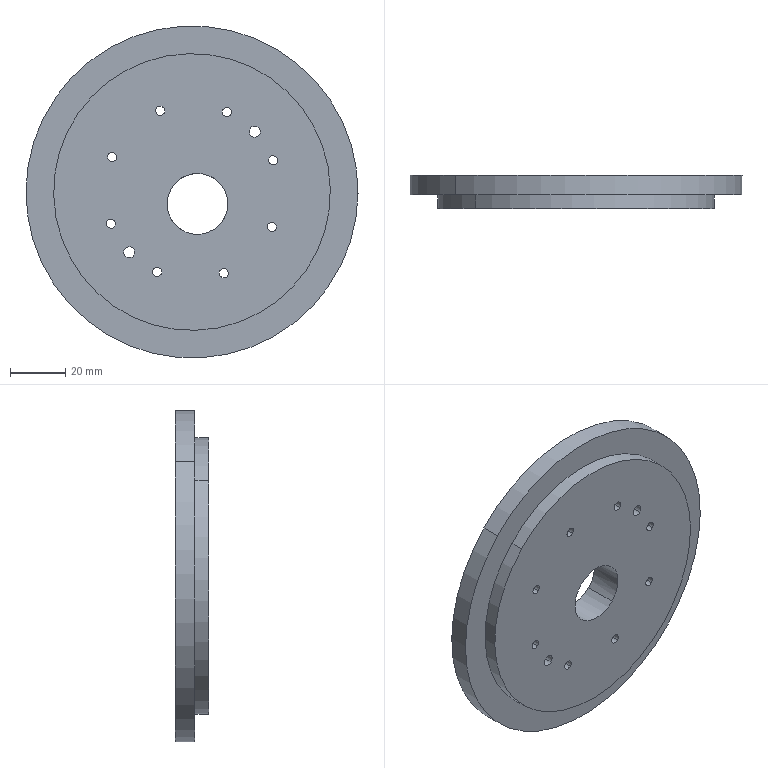Component | SolidWorks | PushRodMotorPlatform-1 | 1 solid | 29 faces | box 120 x 12 x 120 mm | volume 112754 mm3 | cylinder 26 | plane 3 | commonest cylinder face diameters 3.3 x16 4 x4 22 x2 100 x2 120 x2
build123d program:
from build123d import *

# Parameters (mm, degrees)
SKETCH1_2_R             = 60
SKETCH1_2_R_2           = 1.65
SKETCH1_2_R_3           = 2
BOSS_EXTRUDE1_DEPTH     = 12
SKETCH2_R               = 60
SKETCH2_R_2             = 50
CUT_EXTRUDE1_2_DEPTH    = 5
CUT_EXTRUDE1_DEPTH      = 320.099
CUT_EXTRUDE1_DEPTH_BACK = 320.099
SKETCH1_R               = 11


with BuildPart() as part:
    # Sketch1_2 → Boss-Extrude1 (new body)
    with BuildSketch(Plane.XY):
        with Locations((90, 221.39)):
            Circle(SKETCH1_2_R)
        with Locations((118.509, 234.787)):
            Circle(SKETCH1_2_R_2, mode=Mode.SUBTRACT)
        with Locations((119.632, 210.705)):
            Circle(SKETCH1_2_R_2, mode=Mode.SUBTRACT)
        with Locations((103.398, 192.881)):
            Circle(SKETCH1_2_R_2, mode=Mode.SUBTRACT)
        with Locations((91.468, 189.924)):
            Circle(SKETCH1_2_R_3, mode=Mode.SUBTRACT)
        with Locations((79.315, 191.757)):
            Circle(SKETCH1_2_R_2, mode=Mode.SUBTRACT)
        with Locations((61.491, 207.992)):
            Circle(SKETCH1_2_R_2, mode=Mode.SUBTRACT)
        with Locations((60.368, 232.075)):
            Circle(SKETCH1_2_R_2, mode=Mode.SUBTRACT)
        with Locations((76.602, 249.899)):
            Circle(SKETCH1_2_R_2, mode=Mode.SUBTRACT)
        with Locations((88.532, 252.856)):
            Circle(SKETCH1_2_R_3, mode=Mode.SUBTRACT)
        with Locations((100.685, 251.022)):
            Circle(SKETCH1_2_R_2, mode=Mode.SUBTRACT)
    extrude(amount=BOSS_EXTRUDE1_DEPTH)

    # Sketch2 → Cut-Extrude1_2 (cut)
    with BuildSketch(Plane(origin=(0, 0, 0), x_dir=(-1, 0, 0), z_dir=(0, 0, -1))):
        with Locations((-90, 221.39)):
            Circle(SKETCH2_R)
        with Locations((-90, 221.39)):
            Circle(SKETCH2_R_2, mode=Mode.SUBTRACT)
    extrude(amount=-CUT_EXTRUDE1_2_DEPTH, mode=Mode.SUBTRACT)

    # Sketch1 → Cut-Extrude1 (cut, two sides: drawn at the far end of the back side and taken through both)
    with BuildSketch(Plane.XY.offset(-CUT_EXTRUDE1_DEPTH_BACK)):
        with Locations((85.6, 219.613)):
            Circle(SKETCH1_R)
    extrude(amount=CUT_EXTRUDE1_DEPTH + CUT_EXTRUDE1_DEPTH_BACK, mode=Mode.SUBTRACT)


solid = part.part

# Placed as in the assembly
solid = solid.moved(Location((499.474, 964, -2315.533), (-90, 0, -136.538)))
STEP:
#1=COLOUR_RGB('',0.7922,0.8196,0.9333);
#2=FILL_AREA_STYLE_COLOUR('',#1);
#3=FILL_AREA_STYLE('',(#2));
#4=SURFACE_STYLE_FILL_AREA(#3);
#5=SURFACE_SIDE_STYLE('',(#4));
#6=SURFACE_STYLE_USAGE(.BOTH.,#5);
#7=PRESENTATION_STYLE_ASSIGNMENT((#6));
#8=CARTESIAN_POINT('',(23.48,37.953,-82.867));
#9=VERTEX_POINT('',#8);
#10=CARTESIAN_POINT('',(22.851,37.953,-82.271));
#11=VERTEX_POINT('',#10);
#12=CARTESIAN_POINT('',(23.48,37.953,-82.867));
#13=CARTESIAN_POINT('',(23.441,37.953,-82.908));
#14=CARTESIAN_POINT('',(23.395,37.953,-82.941));
#15=CARTESIAN_POINT('',(23.29,37.953,-82.988));
#16=CARTESIAN_POINT('',(23.235,37.953,-83.));
#17=CARTESIAN_POINT('',(23.12,37.953,-83.003));
#18=CARTESIAN_POINT('',(23.064,37.953,-82.994));
#19=CARTESIAN_POINT('',(22.957,37.953,-82.953));
#20=CARTESIAN_POINT('',(22.91,37.953,-82.923));
#21=CARTESIAN_POINT('',(22.826,37.953,-82.844));
#22=CARTESIAN_POINT('',(22.794,37.953,-82.798));
#23=CARTESIAN_POINT('',(22.747,37.953,-82.693));
#24=CARTESIAN_POINT('',(22.734,37.953,-82.638));
#25=CARTESIAN_POINT('',(22.731,37.953,-82.523));
#26=CARTESIAN_POINT('',(22.741,37.953,-82.468));
#27=CARTESIAN_POINT('',(22.782,37.953,-82.36));
#28=CARTESIAN_POINT('',(22.812,37.953,-82.313));
#29=CARTESIAN_POINT('',(22.851,37.953,-82.271));
#30=B_SPLINE_CURVE_WITH_KNOTS('',3,(#12,#13,#14,#15,#16,#17,#18,#19,#20,#21,#22,#23,#24,#25,#26,#27,#28,#29),.UNSPECIFIED.,.F.,.F.,(4,2,2,2,2,2,2,2,4),(0.5,0.5625,0.625,0.6875,0.75,0.8125,0.875,0.9375,1.),.UNSPECIFIED.);
#31=EDGE_CURVE('',#9,#11,#30,.T.);
#32=ORIENTED_EDGE('',*,*,#31,.F.);
#33=CARTESIAN_POINT('',(23.48,38.425,-82.867));
#34=VERTEX_POINT('',#33);
#35=CARTESIAN_POINT('',(23.48,37.953,-82.867));
#36=DIRECTION('',(-0.,1.,0.));
#37=VECTOR('',#36,39.37);
#38=LINE('',#35,#37);
#39=EDGE_CURVE('',#9,#34,#38,.T.);
#40=ORIENTED_EDGE('',*,*,#39,.T.);
#41=CARTESIAN_POINT('',(22.851,38.425,-82.271));
#42=VERTEX_POINT('',#41);
#43=CARTESIAN_POINT('',(23.166,38.425,-82.569));
#44=DIRECTION('',(-0.,1.,0.));
#45=DIRECTION('',(-0.7258,0.,0.6879));
#46=AXIS2_PLACEMENT_3D('',#43,#44,#45);
#47=CIRCLE('',#46,0.4331);
#48=EDGE_CURVE('',#34,#42,#47,.T.);
#49=ORIENTED_EDGE('',*,*,#48,.T.);
#50=CARTESIAN_POINT('',(22.851,37.953,-82.271));
#51=DIRECTION('',(-0.,1.,0.));
#52=VECTOR('',#51,39.37);
#53=LINE('',#50,#52);
#54=EDGE_CURVE('',#11,#42,#53,.T.);
#55=ORIENTED_EDGE('',*,*,#54,.F.);
#56=EDGE_LOOP('',(#32,#40,#49,#55));
#57=FACE_OUTER_BOUND('',#56,.T.);
#58=CARTESIAN_POINT('',(23.166,37.953,-82.569));
#59=DIRECTION('',(-0.,1.,0.));
#60=DIRECTION('',(-0.7258,0.,0.6879));
#61=AXIS2_PLACEMENT_3D('',#58,#59,#60);
#62=CYLINDRICAL_SURFACE('',#61,0.4331);
#63=ADVANCED_FACE('',(#57),#62,.F.);
#64=CARTESIAN_POINT('',(24.517,38.15,-83.753));
#65=VERTEX_POINT('',#64);
#66=CARTESIAN_POINT('',(21.659,38.15,-81.045));
#67=VERTEX_POINT('',#66);
#68=CARTESIAN_POINT('',(23.088,38.15,-82.399));
#69=DIRECTION('',(0.,-1.,-0.));
#70=DIRECTION('',(0.7258,0.,-0.6879));
#71=AXIS2_PLACEMENT_3D('',#68,#69,#70);
#72=CIRCLE('',#71,1.969);
#73=EDGE_CURVE('',#65,#67,#72,.T.);
#74=ORIENTED_EDGE('',*,*,#73,.T.);
#75=CARTESIAN_POINT('',(21.659,37.953,-81.045));
#76=VERTEX_POINT('',#75);
#77=CARTESIAN_POINT('',(21.659,38.15,-81.045));
#78=DIRECTION('',(0.,-1.,-0.));
#79=VECTOR('',#78,39.37);
#80=LINE('',#77,#79);
#81=EDGE_CURVE('',#67,#76,#80,.T.);
#82=ORIENTED_EDGE('',*,*,#81,.T.);
#83=CARTESIAN_POINT('',(24.517,37.953,-83.753));
#84=VERTEX_POINT('',#83);
#85=CARTESIAN_POINT('',(23.088,37.953,-82.399));
#86=DIRECTION('',(0.,-1.,-0.));
#87=DIRECTION('',(0.7258,0.,-0.6879));
#88=AXIS2_PLACEMENT_3D('',#85,#86,#87);
#89=CIRCLE('',#88,1.969);
#90=EDGE_CURVE('',#84,#76,#89,.T.);
#91=ORIENTED_EDGE('',*,*,#90,.F.);
#92=CARTESIAN_POINT('',(24.517,38.15,-83.753));
#93=DIRECTION('',(0.,-1.,-0.));
#94=VECTOR('',#93,39.37);
#95=LINE('',#92,#94);
#96=EDGE_CURVE('',#65,#84,#95,.T.);
#97=ORIENTED_EDGE('',*,*,#96,.F.);
#98=EDGE_LOOP('',(#74,#82,#91,#97));
#99=FACE_OUTER_BOUND('',#98,.T.);
#100=CARTESIAN_POINT('',(23.088,38.15,-82.399));
#101=DIRECTION('',(0.,-1.,-0.));
#102=DIRECTION('',(0.7258,0.,-0.6879));
#103=AXIS2_PLACEMENT_3D('',#100,#101,#102);
#104=CYLINDRICAL_SURFACE('',#103,1.969);
#105=ADVANCED_FACE('',(#99),#104,.T.);
#106=CARTESIAN_POINT('',(23.632,38.425,-81.308));
#107=VERTEX_POINT('',#106);
#108=CARTESIAN_POINT('',(23.538,38.425,-81.218));
#109=VERTEX_POINT('',#108);
#110=CARTESIAN_POINT('',(23.585,38.425,-81.263));
#111=DIRECTION('',(-0.,1.,0.));
#112=DIRECTION('',(-0.7258,0.,0.6879));
#113=AXIS2_PLACEMENT_3D('',#110,#111,#112);
#114=CIRCLE('',#113,0.06496);
#115=EDGE_CURVE('',#107,#109,#114,.T.);
#116=ORIENTED_EDGE('',*,*,#115,.T.);
#117=CARTESIAN_POINT('',(23.538,37.953,-81.218));
#118=VERTEX_POINT('',#117);
#119=CARTESIAN_POINT('',(23.538,38.425,-81.218));
#120=DIRECTION('',(0.,-1.,-0.));
#121=VECTOR('',#120,39.37);
#122=LINE('',#119,#121);
#123=EDGE_CURVE('',#109,#118,#122,.T.);
#124=ORIENTED_EDGE('',*,*,#123,.T.);
#125=CARTESIAN_POINT('',(23.632,37.953,-81.308));
#126=VERTEX_POINT('',#125);
#127=CARTESIAN_POINT('',(23.585,37.953,-81.263));
#128=DIRECTION('',(-0.,1.,0.));
#129=DIRECTION('',(-0.7258,0.,0.6879));
#130=AXIS2_PLACEMENT_3D('',#127,#128,#129);
#131=CIRCLE('',#130,0.06496);
#132=EDGE_CURVE('',#126,#118,#131,.T.);
#133=ORIENTED_EDGE('',*,*,#132,.F.);
#134=CARTESIAN_POINT('',(23.632,38.425,-81.308));
#135=DIRECTION('',(0.,-1.,-0.));
#136=VECTOR('',#135,39.37);
#137=LINE('',#134,#136);
#138=EDGE_CURVE('',#107,#126,#137,.T.);
#139=ORIENTED_EDGE('',*,*,#138,.F.);
#140=EDGE_LOOP('',(#116,#124,#133,#139));
#141=FACE_OUTER_BOUND('',#140,.T.);
#142=CARTESIAN_POINT('',(23.585,38.425,-81.263));
#143=DIRECTION('',(0.,-1.,-0.));
#144=DIRECTION('',(0.7258,0.,-0.6879));
#145=AXIS2_PLACEMENT_3D('',#142,#143,#144);
#146=CYLINDRICAL_SURFACE('',#145,0.06496);
#147=ADVANCED_FACE('',(#141),#146,.F.);
#148=CARTESIAN_POINT('',(24.039,38.425,-81.594));
#149=VERTEX_POINT('',#148);
#150=CARTESIAN_POINT('',(23.925,38.425,-81.485));
#151=VERTEX_POINT('',#150);
#152=CARTESIAN_POINT('',(23.982,38.425,-81.54));
#153=DIRECTION('',(-0.,1.,0.));
#154=DIRECTION('',(-0.7258,0.,0.6879));
#155=AXIS2_PLACEMENT_3D('',#152,#153,#154);
#156=CIRCLE('',#155,0.07874);
#157=EDGE_CURVE('',#149,#151,#156,.T.);
#158=ORIENTED_EDGE('',*,*,#157,.T.);
#159=CARTESIAN_POINT('',(23.925,37.953,-81.485));
#160=VERTEX_POINT('',#159);
#161=CARTESIAN_POINT('',(23.925,38.425,-81.485));
#162=DIRECTION('',(0.,-1.,-0.));
#163=VECTOR('',#162,39.37);
#164=LINE('',#161,#163);
#165=EDGE_CURVE('',#151,#160,#164,.T.);
#166=ORIENTED_EDGE('',*,*,#165,.T.);
#167=CARTESIAN_POINT('',(24.039,37.953,-81.594));
#168=VERTEX_POINT('',#167);
#169=CARTESIAN_POINT('',(23.982,37.953,-81.54));
#170=DIRECTION('',(-0.,1.,0.));
#171=DIRECTION('',(-0.7258,0.,0.6879));
#172=AXIS2_PLACEMENT_3D('',#169,#170,#171);
#173=CIRCLE('',#172,0.07874);
#174=EDGE_CURVE('',#168,#160,#173,.T.);
#175=ORIENTED_EDGE('',*,*,#174,.F.);
#176=CARTESIAN_POINT('',(24.039,38.425,-81.594));
#177=DIRECTION('',(0.,-1.,-0.));
#178=VECTOR('',#177,39.37);
#179=LINE('',#176,#178);
#180=EDGE_CURVE('',#149,#168,#179,.T.);
#181=ORIENTED_EDGE('',*,*,#180,.F.);
#182=EDGE_LOOP('',(#158,#166,#175,#181));
#183=FACE_OUTER_BOUND('',#182,.T.);
#184=CARTESIAN_POINT('',(23.982,38.425,-81.54));
#185=DIRECTION('',(0.,-1.,-0.));
#186=DIRECTION('',(0.7258,0.,-0.6879));
#187=AXIS2_PLACEMENT_3D('',#184,#185,#186);
#188=CYLINDRICAL_SURFACE('',#187,0.07874);
#189=ADVANCED_FACE('',(#183),#188,.F.);
#190=CARTESIAN_POINT('',(24.29,38.425,-81.992));
#191=VERTEX_POINT('',#190);
#192=CARTESIAN_POINT('',(24.196,38.425,-81.902));
#193=VERTEX_POINT('',#192);
#194=CARTESIAN_POINT('',(24.243,38.425,-81.947));
#195=DIRECTION('',(-0.,1.,0.));
#196=DIRECTION('',(-0.7258,0.,0.6879));
#197=AXIS2_PLACEMENT_3D('',#194,#195,#196);
#198=CIRCLE('',#197,0.06496);
#199=EDGE_CURVE('',#191,#193,#198,.T.);
#200=ORIENTED_EDGE('',*,*,#199,.T.);
#201=CARTESIAN_POINT('',(24.196,37.953,-81.902));
#202=VERTEX_POINT('',#201);
#203=CARTESIAN_POINT('',(24.196,38.425,-81.902));
#204=DIRECTION('',(0.,-1.,-0.));
#205=VECTOR('',#204,39.37);
#206=LINE('',#203,#205);
#207=EDGE_CURVE('',#193,#202,#206,.T.);
#208=ORIENTED_EDGE('',*,*,#207,.T.);
#209=CARTESIAN_POINT('',(24.29,37.953,-81.992));
#210=VERTEX_POINT('',#209);
#211=CARTESIAN_POINT('',(24.243,37.953,-81.947));
#212=DIRECTION('',(-0.,1.,0.));
#213=DIRECTION('',(-0.7258,0.,0.6879));
#214=AXIS2_PLACEMENT_3D('',#211,#212,#213);
#215=CIRCLE('',#214,0.06496);
#216=EDGE_CURVE('',#210,#202,#215,.T.);
#217=ORIENTED_EDGE('',*,*,#216,.F.);
#218=CARTESIAN_POINT('',(24.29,38.425,-81.992));
#219=DIRECTION('',(0.,-1.,-0.));
#220=VECTOR('',#219,39.37);
#221=LINE('',#218,#220);
#222=EDGE_CURVE('',#191,#210,#221,.T.);
#223=ORIENTED_EDGE('',*,*,#222,.F.);
#224=EDGE_LOOP('',(#200,#208,#217,#223));
#225=FACE_OUTER_BOUND('',#224,.T.);
#226=CARTESIAN_POINT('',(24.243,38.425,-81.947));
#227=DIRECTION('',(0.,-1.,-0.));
#228=DIRECTION('',(0.7258,0.,-0.6879));
#229=AXIS2_PLACEMENT_3D('',#226,#227,#228);
#230=CYLINDRICAL_SURFACE('',#229,0.06496);
#231=ADVANCED_FACE('',(#225),#230,.F.);
#232=CARTESIAN_POINT('',(24.271,38.425,-82.941));
#233=VERTEX_POINT('',#232);
#234=CARTESIAN_POINT('',(24.177,38.425,-82.851));
#235=VERTEX_POINT('',#234);
#236=CARTESIAN_POINT('',(24.224,38.425,-82.896));
#237=DIRECTION('',(-0.,1.,0.));
#238=DIRECTION('',(-0.7258,0.,0.6879));
#239=AXIS2_PLACEMENT_3D('',#236,#237,#238);
#240=CIRCLE('',#239,0.06496);
#241=EDGE_CURVE('',#233,#235,#240,.T.);
#242=ORIENTED_EDGE('',*,*,#241,.T.);
#243=CARTESIAN_POINT('',(24.177,37.953,-82.851));
#244=VERTEX_POINT('',#243);
#245=CARTESIAN_POINT('',(24.177,38.425,-82.851));
#246=DIRECTION('',(0.,-1.,-0.));
#247=VECTOR('',#246,39.37);
#248=LINE('',#245,#247);
#249=EDGE_CURVE('',#235,#244,#248,.T.);
#250=ORIENTED_EDGE('',*,*,#249,.T.);
#251=CARTESIAN_POINT('',(24.271,37.953,-82.941));
#252=VERTEX_POINT('',#251);
#253=CARTESIAN_POINT('',(24.224,37.953,-82.896));
#254=DIRECTION('',(-0.,1.,0.));
#255=DIRECTION('',(-0.7258,0.,0.6879));
#256=AXIS2_PLACEMENT_3D('',#253,#254,#255);
#257=CIRCLE('',#256,0.06496);
#258=EDGE_CURVE('',#252,#244,#257,.T.);
#259=ORIENTED_EDGE('',*,*,#258,.F.);
#260=CARTESIAN_POINT('',(24.271,38.425,-82.941));
#261=DIRECTION('',(0.,-1.,-0.));
#262=VECTOR('',#261,39.37);
#263=LINE('',#260,#262);
#264=EDGE_CURVE('',#233,#252,#263,.T.);
#265=ORIENTED_EDGE('',*,*,#264,.F.);
#266=EDGE_LOOP('',(#242,#250,#259,#265));
#267=FACE_OUTER_BOUND('',#266,.T.);
#268=CARTESIAN_POINT('',(24.224,38.425,-82.896));
#269=DIRECTION('',(0.,-1.,-0.));
#270=DIRECTION('',(0.7258,0.,-0.6879));
#271=AXIS2_PLACEMENT_3D('',#268,#269,#270);
#272=CYLINDRICAL_SURFACE('',#271,0.06496);
#273=ADVANCED_FACE('',(#267),#272,.F.);
#274=CARTESIAN_POINT('',(23.587,38.425,-83.599));
#275=VERTEX_POINT('',#274);
#276=CARTESIAN_POINT('',(23.493,38.425,-83.509));
#277=VERTEX_POINT('',#276);
#278=CARTESIAN_POINT('',(23.54,38.425,-83.554));
#279=DIRECTION('',(-0.,1.,0.));
#280=DIRECTION('',(-0.7258,0.,0.6879));
#281=AXIS2_PLACEMENT_3D('',#278,#279,#280);
#282=CIRCLE('',#281,0.06496);
#283=EDGE_CURVE('',#275,#277,#282,.T.);
#284=ORIENTED_EDGE('',*,*,#283,.T.);
#285=CARTESIAN_POINT('',(23.493,37.953,-83.509));
#286=VERTEX_POINT('',#285);
#287=CARTESIAN_POINT('',(23.493,38.425,-83.509));
#288=DIRECTION('',(0.,-1.,-0.));
#289=VECTOR('',#288,39.37);
#290=LINE('',#287,#289);
#291=EDGE_CURVE('',#277,#286,#290,.T.);
#292=ORIENTED_EDGE('',*,*,#291,.T.);
#293=CARTESIAN_POINT('',(23.587,37.953,-83.599));
#294=VERTEX_POINT('',#293);
#295=CARTESIAN_POINT('',(23.54,37.953,-83.554));
#296=DIRECTION('',(-0.,1.,0.));
#297=DIRECTION('',(-0.7258,0.,0.6879));
#298=AXIS2_PLACEMENT_3D('',#295,#296,#297);
#299=CIRCLE('',#298,0.06496);
#300=EDGE_CURVE('',#294,#286,#299,.T.);
#301=ORIENTED_EDGE('',*,*,#300,.F.);
#302=CARTESIAN_POINT('',(23.587,38.425,-83.599));
#303=DIRECTION('',(0.,-1.,-0.));
#304=VECTOR('',#303,39.37);
#305=LINE('',#302,#304);
#306=EDGE_CURVE('',#275,#294,#305,.T.);
#307=ORIENTED_EDGE('',*,*,#306,.F.);
#308=EDGE_LOOP('',(#284,#292,#301,#307));
#309=FACE_OUTER_BOUND('',#308,.T.);
#310=CARTESIAN_POINT('',(23.54,38.425,-83.554));
#311=DIRECTION('',(0.,-1.,-0.));
#312=DIRECTION('',(0.7258,0.,-0.6879));
#313=AXIS2_PLACEMENT_3D('',#310,#311,#312);
#314=CYLINDRICAL_SURFACE('',#313,0.06496);
#315=ADVANCED_FACE('',(#309),#314,.F.);
#316=CARTESIAN_POINT('',(22.638,38.425,-83.58));
#317=VERTEX_POINT('',#316);
#318=CARTESIAN_POINT('',(22.544,38.425,-83.49));
#319=VERTEX_POINT('',#318);
#320=CARTESIAN_POINT('',(22.591,38.425,-83.535));
#321=DIRECTION('',(-0.,1.,0.));
#322=DIRECTION('',(-0.7258,0.,0.6879));
#323=AXIS2_PLACEMENT_3D('',#320,#321,#322);
#324=CIRCLE('',#323,0.06496);
#325=EDGE_CURVE('',#317,#319,#324,.T.);
#326=ORIENTED_EDGE('',*,*,#325,.T.);
#327=CARTESIAN_POINT('',(22.544,37.953,-83.49));
#328=VERTEX_POINT('',#327);
#329=CARTESIAN_POINT('',(22.544,38.425,-83.49));
#330=DIRECTION('',(0.,-1.,-0.));
#331=VECTOR('',#330,39.37);
#332=LINE('',#329,#331);
#333=EDGE_CURVE('',#319,#328,#332,.T.);
#334=ORIENTED_EDGE('',*,*,#333,.T.);
#335=CARTESIAN_POINT('',(22.638,37.953,-83.58));
#336=VERTEX_POINT('',#335);
#337=CARTESIAN_POINT('',(22.591,37.953,-83.535));
#338=DIRECTION('',(-0.,1.,0.));
#339=DIRECTION('',(-0.7258,0.,0.6879));
#340=AXIS2_PLACEMENT_3D('',#337,#338,#339);
#341=CIRCLE('',#340,0.06496);
#342=EDGE_CURVE('',#336,#328,#341,.T.);
#343=ORIENTED_EDGE('',*,*,#342,.F.);
#344=CARTESIAN_POINT('',(22.638,38.425,-83.58));
#345=DIRECTION('',(0.,-1.,-0.));
#346=VECTOR('',#345,39.37);
#347=LINE('',#344,#346);
#348=EDGE_CURVE('',#317,#336,#347,.T.);
#349=ORIENTED_EDGE('',*,*,#348,.F.);
#350=EDGE_LOOP('',(#326,#334,#343,#349));
#351=FACE_OUTER_BOUND('',#350,.T.);
#352=CARTESIAN_POINT('',(22.591,38.425,-83.535));
#353=DIRECTION('',(0.,-1.,-0.));
#354=DIRECTION('',(0.7258,0.,-0.6879));
#355=AXIS2_PLACEMENT_3D('',#352,#353,#354);
#356=CYLINDRICAL_SURFACE('',#355,0.06496);
#357=ADVANCED_FACE('',(#351),#356,.F.);
#358=CARTESIAN_POINT('',(22.251,38.425,-83.313));
#359=VERTEX_POINT('',#358);
#360=CARTESIAN_POINT('',(22.137,38.425,-83.204));
#361=VERTEX_POINT('',#360);
#362=CARTESIAN_POINT('',(22.194,38.425,-83.258));
#363=DIRECTION('',(-0.,1.,0.));
#364=DIRECTION('',(-0.7258,0.,0.6879));
#365=AXIS2_PLACEMENT_3D('',#362,#363,#364);
#366=CIRCLE('',#365,0.07874);
#367=EDGE_CURVE('',#359,#361,#366,.T.);
#368=ORIENTED_EDGE('',*,*,#367,.T.);
#369=CARTESIAN_POINT('',(22.137,37.953,-83.204));
#370=VERTEX_POINT('',#369);
#371=CARTESIAN_POINT('',(22.137,38.425,-83.204));
#372=DIRECTION('',(0.,-1.,-0.));
#373=VECTOR('',#372,39.37);
#374=LINE('',#371,#373);
#375=EDGE_CURVE('',#361,#370,#374,.T.);
#376=ORIENTED_EDGE('',*,*,#375,.T.);
#377=CARTESIAN_POINT('',(22.251,37.953,-83.313));
#378=VERTEX_POINT('',#377);
#379=CARTESIAN_POINT('',(22.194,37.953,-83.258));
#380=DIRECTION('',(-0.,1.,0.));
#381=DIRECTION('',(-0.7258,0.,0.6879));
#382=AXIS2_PLACEMENT_3D('',#379,#380,#381);
#383=CIRCLE('',#382,0.07874);
#384=EDGE_CURVE('',#378,#370,#383,.T.);
#385=ORIENTED_EDGE('',*,*,#384,.F.);
#386=CARTESIAN_POINT('',(22.251,38.425,-83.313));
#387=DIRECTION('',(0.,-1.,-0.));
#388=VECTOR('',#387,39.37);
#389=LINE('',#386,#388);
#390=EDGE_CURVE('',#359,#378,#389,.T.);
#391=ORIENTED_EDGE('',*,*,#390,.F.);
#392=EDGE_LOOP('',(#368,#376,#385,#391));
#393=FACE_OUTER_BOUND('',#392,.T.);
#394=CARTESIAN_POINT('',(22.194,38.425,-83.258));
#395=DIRECTION('',(0.,-1.,-0.));
#396=DIRECTION('',(0.7258,0.,-0.6879));
#397=AXIS2_PLACEMENT_3D('',#394,#395,#396);
#398=CYLINDRICAL_SURFACE('',#397,0.07874);
#399=ADVANCED_FACE('',(#393),#398,.F.);
#400=CARTESIAN_POINT('',(21.98,38.425,-82.895));
#401=VERTEX_POINT('',#400);
#402=CARTESIAN_POINT('',(21.886,38.425,-82.806));
#403=VERTEX_POINT('',#402);
#404=CARTESIAN_POINT('',(21.933,38.425,-82.851));
#405=DIRECTION('',(-0.,1.,0.));
#406=DIRECTION('',(-0.7258,0.,0.6879));
#407=AXIS2_PLACEMENT_3D('',#404,#405,#406);
#408=CIRCLE('',#407,0.06496);
#409=EDGE_CURVE('',#401,#403,#408,.T.);
#410=ORIENTED_EDGE('',*,*,#409,.T.);
#411=CARTESIAN_POINT('',(21.886,37.953,-82.806));
#412=VERTEX_POINT('',#411);
#413=CARTESIAN_POINT('',(21.886,38.425,-82.806));
#414=DIRECTION('',(0.,-1.,-0.));
#415=VECTOR('',#414,39.37);
#416=LINE('',#413,#415);
#417=EDGE_CURVE('',#403,#412,#416,.T.);
#418=ORIENTED_EDGE('',*,*,#417,.T.);
#419=CARTESIAN_POINT('',(21.98,37.953,-82.895));
#420=VERTEX_POINT('',#419);
#421=CARTESIAN_POINT('',(21.933,37.953,-82.851));
#422=DIRECTION('',(-0.,1.,0.));
#423=DIRECTION('',(-0.7258,0.,0.6879));
#424=AXIS2_PLACEMENT_3D('',#421,#422,#423);
#425=CIRCLE('',#424,0.06496);
#426=EDGE_CURVE('',#420,#412,#425,.T.);
#427=ORIENTED_EDGE('',*,*,#426,.F.);
#428=CARTESIAN_POINT('',(21.98,38.425,-82.895));
#429=DIRECTION('',(0.,-1.,-0.));
#430=VECTOR('',#429,39.37);
#431=LINE('',#428,#430);
#432=EDGE_CURVE('',#401,#420,#431,.T.);
#433=ORIENTED_EDGE('',*,*,#432,.F.);
#434=EDGE_LOOP('',(#410,#418,#427,#433));
#435=FACE_OUTER_BOUND('',#434,.T.);
#436=CARTESIAN_POINT('',(21.933,38.425,-82.851));
#437=DIRECTION('',(0.,-1.,-0.));
#438=DIRECTION('',(0.7258,0.,-0.6879));
#439=AXIS2_PLACEMENT_3D('',#436,#437,#438);
#440=CYLINDRICAL_SURFACE('',#439,0.06496);
#441=ADVANCED_FACE('',(#435),#440,.F.);
#442=CARTESIAN_POINT('',(21.999,38.425,-81.946));
#443=VERTEX_POINT('',#442);
#444=CARTESIAN_POINT('',(21.905,38.425,-81.857));
#445=VERTEX_POINT('',#444);
#446=CARTESIAN_POINT('',(21.952,38.425,-81.902));
#447=DIRECTION('',(-0.,1.,0.));
#448=DIRECTION('',(-0.7258,0.,0.6879));
#449=AXIS2_PLACEMENT_3D('',#446,#447,#448);
#450=CIRCLE('',#449,0.06496);
#451=EDGE_CURVE('',#443,#445,#450,.T.);
#452=ORIENTED_EDGE('',*,*,#451,.T.);
#453=CARTESIAN_POINT('',(21.905,37.953,-81.857));
#454=VERTEX_POINT('',#453);
#455=CARTESIAN_POINT('',(21.905,38.425,-81.857));
#456=DIRECTION('',(0.,-1.,-0.));
#457=VECTOR('',#456,39.37);
#458=LINE('',#455,#457);
#459=EDGE_CURVE('',#445,#454,#458,.T.);
#460=ORIENTED_EDGE('',*,*,#459,.T.);
#461=CARTESIAN_POINT('',(21.999,37.953,-81.946));
#462=VERTEX_POINT('',#461);
#463=CARTESIAN_POINT('',(21.952,37.953,-81.902));
#464=DIRECTION('',(-0.,1.,0.));
#465=DIRECTION('',(-0.7258,0.,0.6879));
#466=AXIS2_PLACEMENT_3D('',#463,#464,#465);
#467=CIRCLE('',#466,0.06496);
#468=EDGE_CURVE('',#462,#454,#467,.T.);
#469=ORIENTED_EDGE('',*,*,#468,.F.);
#470=CARTESIAN_POINT('',(21.999,38.425,-81.946));
#471=DIRECTION('',(0.,-1.,-0.));
#472=VECTOR('',#471,39.37);
#473=LINE('',#470,#472);
#474=EDGE_CURVE('',#443,#462,#473,.T.);
#475=ORIENTED_EDGE('',*,*,#474,.F.);
#476=EDGE_LOOP('',(#452,#460,#469,#475));
#477=FACE_OUTER_BOUND('',#476,.T.);
#478=CARTESIAN_POINT('',(21.952,38.425,-81.902));
#479=DIRECTION('',(0.,-1.,-0.));
#480=DIRECTION('',(0.7258,0.,-0.6879));
#481=AXIS2_PLACEMENT_3D('',#478,#479,#480);
#482=CYLINDRICAL_SURFACE('',#481,0.06496);
#483=ADVANCED_FACE('',(#477),#482,.F.);
#484=CARTESIAN_POINT('',(22.683,38.425,-81.289));
#485=VERTEX_POINT('',#484);
#486=CARTESIAN_POINT('',(22.589,38.425,-81.199));
#487=VERTEX_POINT('',#486);
#488=CARTESIAN_POINT('',(22.636,38.425,-81.244));
#489=DIRECTION('',(-0.,1.,0.));
#490=DIRECTION('',(-0.7258,0.,0.6879));
#491=AXIS2_PLACEMENT_3D('',#488,#489,#490);
#492=CIRCLE('',#491,0.06496);
#493=EDGE_CURVE('',#485,#487,#492,.T.);
#494=ORIENTED_EDGE('',*,*,#493,.T.);
#495=CARTESIAN_POINT('',(22.589,37.953,-81.199));
#496=VERTEX_POINT('',#495);
#497=CARTESIAN_POINT('',(22.589,38.425,-81.199));
#498=DIRECTION('',(0.,-1.,-0.));
#499=VECTOR('',#498,39.37);
#500=LINE('',#497,#499);
#501=EDGE_CURVE('',#487,#496,#500,.T.);
#502=ORIENTED_EDGE('',*,*,#501,.T.);
#503=CARTESIAN_POINT('',(22.683,37.953,-81.289));
#504=VERTEX_POINT('',#503);
#505=CARTESIAN_POINT('',(22.636,37.953,-81.244));
#506=DIRECTION('',(-0.,1.,0.));
#507=DIRECTION('',(-0.7258,0.,0.6879));
#508=AXIS2_PLACEMENT_3D('',#505,#506,#507);
#509=CIRCLE('',#508,0.06496);
#510=EDGE_CURVE('',#504,#496,#509,.T.);
#511=ORIENTED_EDGE('',*,*,#510,.F.);
#512=CARTESIAN_POINT('',(22.683,38.425,-81.289));
#513=DIRECTION('',(0.,-1.,-0.));
#514=VECTOR('',#513,39.37);
#515=LINE('',#512,#514);
#516=EDGE_CURVE('',#485,#504,#515,.T.);
#517=ORIENTED_EDGE('',*,*,#516,.F.);
#518=EDGE_LOOP('',(#494,#502,#511,#517));
#519=FACE_OUTER_BOUND('',#518,.T.);
#520=CARTESIAN_POINT('',(22.636,38.425,-81.244));
#521=DIRECTION('',(0.,-1.,-0.));
#522=DIRECTION('',(0.7258,0.,-0.6879));
#523=AXIS2_PLACEMENT_3D('',#520,#521,#522);
#524=CYLINDRICAL_SURFACE('',#523,0.06496);
#525=ADVANCED_FACE('',(#519),#524,.F.);
#526=CARTESIAN_POINT('',(21.374,38.425,-80.774));
#527=VERTEX_POINT('',#526);
#528=CARTESIAN_POINT('',(24.803,38.425,-84.024));
#529=VERTEX_POINT('',#528);
#530=CARTESIAN_POINT('',(23.088,38.425,-82.399));
#531=DIRECTION('',(-0.,1.,0.));
#532=DIRECTION('',(-0.7258,-0.,0.6879));
#533=AXIS2_PLACEMENT_3D('',#530,#531,#532);
#534=CIRCLE('',#533,2.362);
#535=EDGE_CURVE('',#527,#529,#534,.T.);
#536=ORIENTED_EDGE('',*,*,#535,.F.);
#537=CARTESIAN_POINT('',(21.374,38.15,-80.774));
#538=VERTEX_POINT('',#537);
#539=CARTESIAN_POINT('',(21.374,38.425,-80.774));
#540=DIRECTION('',(0.,-1.,-0.));
#541=VECTOR('',#540,39.37);
#542=LINE('',#539,#541);
#543=EDGE_CURVE('',#527,#538,#542,.T.);
#544=ORIENTED_EDGE('',*,*,#543,.T.);
#545=CARTESIAN_POINT('',(24.803,38.15,-84.024));
#546=VERTEX_POINT('',#545);
#547=CARTESIAN_POINT('',(23.088,38.15,-82.399));
#548=DIRECTION('',(0.,-1.,-0.));
#549=DIRECTION('',(0.7258,0.,-0.6879));
#550=AXIS2_PLACEMENT_3D('',#547,#548,#549);
#551=CIRCLE('',#550,2.362);
#552=EDGE_CURVE('',#546,#538,#551,.T.);
#553=ORIENTED_EDGE('',*,*,#552,.F.);
#554=CARTESIAN_POINT('',(24.803,38.425,-84.024));
#555=DIRECTION('',(0.,-1.,-0.));
#556=VECTOR('',#555,39.37);
#557=LINE('',#554,#556);
#558=EDGE_CURVE('',#529,#546,#557,.T.);
#559=ORIENTED_EDGE('',*,*,#558,.F.);
#560=EDGE_LOOP('',(#536,#544,#553,#559));
#561=FACE_OUTER_BOUND('',#560,.T.);
#562=CARTESIAN_POINT('',(23.088,38.425,-82.399));
#563=DIRECTION('',(0.,-1.,-0.));
#564=DIRECTION('',(0.7258,0.,-0.6879));
#565=AXIS2_PLACEMENT_3D('',#562,#563,#564);
#566=CYLINDRICAL_SURFACE('',#565,2.362);
#567=ADVANCED_FACE('',(#561),#566,.T.);
#568=CARTESIAN_POINT('',(22.851,37.953,-82.271));
#569=CARTESIAN_POINT('',(22.891,37.953,-82.229));
#570=CARTESIAN_POINT('',(22.937,37.953,-82.197));
#571=CARTESIAN_POINT('',(23.042,37.953,-82.15));
#572=CARTESIAN_POINT('',(23.097,37.953,-82.138));
#573=CARTESIAN_POINT('',(23.212,37.953,-82.134));
#574=CARTESIAN_POINT('',(23.267,37.953,-82.144));
#575=CARTESIAN_POINT('',(23.374,37.953,-82.185));
#576=CARTESIAN_POINT('',(23.422,37.953,-82.215));
#577=CARTESIAN_POINT('',(23.505,37.953,-82.294));
#578=CARTESIAN_POINT('',(23.538,37.953,-82.34));
#579=CARTESIAN_POINT('',(23.585,37.953,-82.445));
#580=CARTESIAN_POINT('',(23.597,37.953,-82.5));
#581=CARTESIAN_POINT('',(23.6,37.953,-82.615));
#582=CARTESIAN_POINT('',(23.591,37.953,-82.67));
#583=CARTESIAN_POINT('',(23.55,37.953,-82.777));
#584=CARTESIAN_POINT('',(23.52,37.953,-82.825));
#585=CARTESIAN_POINT('',(23.48,37.953,-82.867));
#586=B_SPLINE_CURVE_WITH_KNOTS('',3,(#568,#569,#570,#571,#572,#573,#574,#575,#576,#577,#578,#579,#580,#581,#582,#583,#584,#585),.UNSPECIFIED.,.F.,.F.,(4,2,2,2,2,2,2,2,4),(-0.,0.0625,0.125,0.1875,0.25,0.3125,0.375,0.4375,0.5),.UNSPECIFIED.);
#587=EDGE_CURVE('',#11,#9,#586,.T.);
#588=ORIENTED_EDGE('',*,*,#587,.T.);
#589=ORIENTED_EDGE('',*,*,#31,.T.);
#590=EDGE_LOOP('',(#588,#589));
#591=FACE_BOUND('',#590,.T.);
#592=ORIENTED_EDGE('',*,*,#132,.T.);
#593=CARTESIAN_POINT('',(23.585,37.953,-81.263));
#594=DIRECTION('',(-0.,1.,0.));
#595=DIRECTION('',(-0.7258,0.,0.6879));
#596=AXIS2_PLACEMENT_3D('',#593,#594,#595);
#597=CIRCLE('',#596,0.06496);
#598=EDGE_CURVE('',#118,#126,#597,.T.);
#599=ORIENTED_EDGE('',*,*,#598,.T.);
#600=EDGE_LOOP('',(#592,#599));
#601=FACE_BOUND('',#600,.T.);
#602=ORIENTED_EDGE('',*,*,#174,.T.);
#603=CARTESIAN_POINT('',(23.982,37.953,-81.54));
#604=DIRECTION('',(-0.,1.,0.));
#605=DIRECTION('',(-0.7258,0.,0.6879));
#606=AXIS2_PLACEMENT_3D('',#603,#604,#605);
#607=CIRCLE('',#606,0.07874);
#608=EDGE_CURVE('',#160,#168,#607,.T.);
#609=ORIENTED_EDGE('',*,*,#608,.T.);
#610=EDGE_LOOP('',(#602,#609));
#611=FACE_BOUND('',#610,.T.);
#612=ORIENTED_EDGE('',*,*,#216,.T.);
#613=CARTESIAN_POINT('',(24.243,37.953,-81.947));
#614=DIRECTION('',(-0.,1.,0.));
#615=DIRECTION('',(-0.7258,0.,0.6879));
#616=AXIS2_PLACEMENT_3D('',#613,#614,#615);
#617=CIRCLE('',#616,0.06496);
#618=EDGE_CURVE('',#202,#210,#617,.T.);
#619=ORIENTED_EDGE('',*,*,#618,.T.);
#620=EDGE_LOOP('',(#612,#619));
#621=FACE_BOUND('',#620,.T.);
#622=ORIENTED_EDGE('',*,*,#258,.T.);
#623=CARTESIAN_POINT('',(24.224,37.953,-82.896));
#624=DIRECTION('',(-0.,1.,0.));
#625=DIRECTION('',(-0.7258,0.,0.6879));
#626=AXIS2_PLACEMENT_3D('',#623,#624,#625);
#627=CIRCLE('',#626,0.06496);
#628=EDGE_CURVE('',#244,#252,#627,.T.);
#629=ORIENTED_EDGE('',*,*,#628,.T.);
#630=EDGE_LOOP('',(#622,#629));
#631=FACE_BOUND('',#630,.T.);
#632=ORIENTED_EDGE('',*,*,#300,.T.);
#633=CARTESIAN_POINT('',(23.54,37.953,-83.554));
#634=DIRECTION('',(-0.,1.,0.));
#635=DIRECTION('',(-0.7258,0.,0.6879));
#636=AXIS2_PLACEMENT_3D('',#633,#634,#635);
#637=CIRCLE('',#636,0.06496);
#638=EDGE_CURVE('',#286,#294,#637,.T.);
#639=ORIENTED_EDGE('',*,*,#638,.T.);
#640=EDGE_LOOP('',(#632,#639));
#641=FACE_BOUND('',#640,.T.);
#642=ORIENTED_EDGE('',*,*,#342,.T.);
#643=CARTESIAN_POINT('',(22.591,37.953,-83.535));
#644=DIRECTION('',(-0.,1.,0.));
#645=DIRECTION('',(-0.7258,0.,0.6879));
#646=AXIS2_PLACEMENT_3D('',#643,#644,#645);
#647=CIRCLE('',#646,0.06496);
#648=EDGE_CURVE('',#328,#336,#647,.T.);
#649=ORIENTED_EDGE('',*,*,#648,.T.);
#650=EDGE_LOOP('',(#642,#649));
#651=FACE_BOUND('',#650,.T.);
#652=ORIENTED_EDGE('',*,*,#384,.T.);
#653=CARTESIAN_POINT('',(22.194,37.953,-83.258));
#654=DIRECTION('',(-0.,1.,0.));
#655=DIRECTION('',(-0.7258,0.,0.6879));
#656=AXIS2_PLACEMENT_3D('',#653,#654,#655);
#657=CIRCLE('',#656,0.07874);
#658=EDGE_CURVE('',#370,#378,#657,.T.);
#659=ORIENTED_EDGE('',*,*,#658,.T.);
#660=EDGE_LOOP('',(#652,#659));
#661=FACE_BOUND('',#660,.T.);
#662=ORIENTED_EDGE('',*,*,#426,.T.);
#663=CARTESIAN_POINT('',(21.933,37.953,-82.851));
#664=DIRECTION('',(-0.,1.,0.));
#665=DIRECTION('',(-0.7258,0.,0.6879));
#666=AXIS2_PLACEMENT_3D('',#663,#664,#665);
#667=CIRCLE('',#666,0.06496);
#668=EDGE_CURVE('',#412,#420,#667,.T.);
#669=ORIENTED_EDGE('',*,*,#668,.T.);
#670=EDGE_LOOP('',(#662,#669));
#671=FACE_BOUND('',#670,.T.);
#672=ORIENTED_EDGE('',*,*,#468,.T.);
#673=CARTESIAN_POINT('',(21.952,37.953,-81.902));
#674=DIRECTION('',(-0.,1.,0.));
#675=DIRECTION('',(-0.7258,0.,0.6879));
#676=AXIS2_PLACEMENT_3D('',#673,#674,#675);
#677=CIRCLE('',#676,0.06496);
#678=EDGE_CURVE('',#454,#462,#677,.T.);
#679=ORIENTED_EDGE('',*,*,#678,.T.);
#680=EDGE_LOOP('',(#672,#679));
#681=FACE_BOUND('',#680,.T.);
#682=ORIENTED_EDGE('',*,*,#510,.T.);
#683=CARTESIAN_POINT('',(22.636,37.953,-81.244));
#684=DIRECTION('',(-0.,1.,0.));
#685=DIRECTION('',(-0.7258,0.,0.6879));
#686=AXIS2_PLACEMENT_3D('',#683,#684,#685);
#687=CIRCLE('',#686,0.06496);
#688=EDGE_CURVE('',#496,#504,#687,.T.);
#689=ORIENTED_EDGE('',*,*,#688,.T.);
#690=EDGE_LOOP('',(#682,#689));
#691=FACE_BOUND('',#690,.T.);
#692=ORIENTED_EDGE('',*,*,#90,.T.);
#693=CARTESIAN_POINT('',(23.088,37.953,-82.399));
#694=DIRECTION('',(0.,-1.,-0.));
#695=DIRECTION('',(0.7258,0.,-0.6879));
#696=AXIS2_PLACEMENT_3D('',#693,#694,#695);
#697=CIRCLE('',#696,1.969);
#698=EDGE_CURVE('',#76,#84,#697,.T.);
#699=ORIENTED_EDGE('',*,*,#698,.T.);
#700=EDGE_LOOP('',(#692,#699));
#701=FACE_OUTER_BOUND('',#700,.T.);
#702=CARTESIAN_POINT('',(23.088,37.953,-82.399));
#703=DIRECTION('',(-0.,1.,0.));
#704=DIRECTION('',(-0.7258,-0.,0.6879));
#705=AXIS2_PLACEMENT_3D('',#702,#703,#704);
#706=PLANE('',#705);
#707=ADVANCED_FACE('',(#591,#601,#611,#621,#631,#641,#651,#661,#671,#681,#691,#701),#706,.F.);
#708=ORIENTED_EDGE('',*,*,#543,.F.);
#709=CARTESIAN_POINT('',(23.088,38.425,-82.399));
#710=DIRECTION('',(-0.,1.,0.));
#711=DIRECTION('',(-0.7258,-0.,0.6879));
#712=AXIS2_PLACEMENT_3D('',#709,#710,#711);
#713=CIRCLE('',#712,2.362);
#714=EDGE_CURVE('',#529,#527,#713,.T.);
#715=ORIENTED_EDGE('',*,*,#714,.F.);
#716=ORIENTED_EDGE('',*,*,#558,.T.);
#717=CARTESIAN_POINT('',(23.088,38.15,-82.399));
#718=DIRECTION('',(0.,-1.,-0.));
#719=DIRECTION('',(0.7258,0.,-0.6879));
#720=AXIS2_PLACEMENT_3D('',#717,#718,#719);
#721=CIRCLE('',#720,2.362);
#722=EDGE_CURVE('',#538,#546,#721,.T.);
#723=ORIENTED_EDGE('',*,*,#722,.F.);
#724=EDGE_LOOP('',(#708,#715,#716,#723));
#725=FACE_OUTER_BOUND('',#724,.T.);
#726=CARTESIAN_POINT('',(23.088,38.425,-82.399));
#727=DIRECTION('',(0.,-1.,-0.));
#728=DIRECTION('',(0.7258,0.,-0.6879));
#729=AXIS2_PLACEMENT_3D('',#726,#727,#728);
#730=CYLINDRICAL_SURFACE('',#729,2.362);
#731=ADVANCED_FACE('',(#725),#730,.T.);
#732=CARTESIAN_POINT('',(23.166,38.425,-82.569));
#733=DIRECTION('',(-0.,1.,0.));
#734=DIRECTION('',(-0.7258,0.,0.6879));
#735=AXIS2_PLACEMENT_3D('',#732,#733,#734);
#736=CIRCLE('',#735,0.4331);
#737=EDGE_CURVE('',#42,#34,#736,.T.);
#738=ORIENTED_EDGE('',*,*,#737,.F.);
#739=ORIENTED_EDGE('',*,*,#48,.F.);
#740=EDGE_LOOP('',(#738,#739));
#741=FACE_BOUND('',#740,.T.);
#742=ORIENTED_EDGE('',*,*,#157,.F.);
#743=CARTESIAN_POINT('',(23.982,38.425,-81.54));
#744=DIRECTION('',(-0.,1.,0.));
#745=DIRECTION('',(-0.7258,0.,0.6879));
#746=AXIS2_PLACEMENT_3D('',#743,#744,#745);
#747=CIRCLE('',#746,0.07874);
#748=EDGE_CURVE('',#151,#149,#747,.T.);
#749=ORIENTED_EDGE('',*,*,#748,.F.);
#750=EDGE_LOOP('',(#742,#749));
#751=FACE_BOUND('',#750,.T.);
#752=ORIENTED_EDGE('',*,*,#241,.F.);
#753=CARTESIAN_POINT('',(24.224,38.425,-82.896));
#754=DIRECTION('',(-0.,1.,0.));
#755=DIRECTION('',(-0.7258,0.,0.6879));
#756=AXIS2_PLACEMENT_3D('',#753,#754,#755);
#757=CIRCLE('',#756,0.06496);
#758=EDGE_CURVE('',#235,#233,#757,.T.);
#759=ORIENTED_EDGE('',*,*,#758,.F.);
#760=EDGE_LOOP('',(#752,#759));
#761=FACE_BOUND('',#760,.T.);
#762=ORIENTED_EDGE('',*,*,#325,.F.);
#763=CARTESIAN_POINT('',(22.591,38.425,-83.535));
#764=DIRECTION('',(-0.,1.,0.));
#765=DIRECTION('',(-0.7258,0.,0.6879));
#766=AXIS2_PLACEMENT_3D('',#763,#764,#765);
#767=CIRCLE('',#766,0.06496);
#768=EDGE_CURVE('',#319,#317,#767,.T.);
#769=ORIENTED_EDGE('',*,*,#768,.F.);
#770=EDGE_LOOP('',(#762,#769));
#771=FACE_BOUND('',#770,.T.);
#772=ORIENTED_EDGE('',*,*,#409,.F.);
#773=CARTESIAN_POINT('',(21.933,38.425,-82.851));
#774=DIRECTION('',(-0.,1.,0.));
#775=DIRECTION('',(-0.7258,0.,0.6879));
#776=AXIS2_PLACEMENT_3D('',#773,#774,#775);
#777=CIRCLE('',#776,0.06496);
#778=EDGE_CURVE('',#403,#401,#777,.T.);
#779=ORIENTED_EDGE('',*,*,#778,.F.);
#780=EDGE_LOOP('',(#772,#779));
#781=FACE_BOUND('',#780,.T.);
#782=ORIENTED_EDGE('',*,*,#493,.F.);
#783=CARTESIAN_POINT('',(22.636,38.425,-81.244));
#784=DIRECTION('',(-0.,1.,0.));
#785=DIRECTION('',(-0.7258,0.,0.6879));
#786=AXIS2_PLACEMENT_3D('',#783,#784,#785);
#787=CIRCLE('',#786,0.06496);
#788=EDGE_CURVE('',#487,#485,#787,.T.);
#789=ORIENTED_EDGE('',*,*,#788,.F.);
#790=EDGE_LOOP('',(#782,#789));
#791=FACE_BOUND('',#790,.T.);
#792=ORIENTED_EDGE('',*,*,#714,.T.);
#793=ORIENTED_EDGE('',*,*,#535,.T.);
#794=EDGE_LOOP('',(#792,#793));
#795=FACE_OUTER_BOUND('',#794,.T.);
#796=ORIENTED_EDGE('',*,*,#451,.F.);
#797=CARTESIAN_POINT('',(21.952,38.425,-81.902));
#798=DIRECTION('',(-0.,1.,0.));
#799=DIRECTION('',(-0.7258,0.,0.6879));
#800=AXIS2_PLACEMENT_3D('',#797,#798,#799);
#801=CIRCLE('',#800,0.06496);
#802=EDGE_CURVE('',#445,#443,#801,.T.);
#803=ORIENTED_EDGE('',*,*,#802,.F.);
#804=EDGE_LOOP('',(#796,#803));
#805=FACE_BOUND('',#804,.T.);
#806=ORIENTED_EDGE('',*,*,#367,.F.);
#807=CARTESIAN_POINT('',(22.194,38.425,-83.258));
#808=DIRECTION('',(-0.,1.,0.));
#809=DIRECTION('',(-0.7258,0.,0.6879));
#810=AXIS2_PLACEMENT_3D('',#807,#808,#809);
#811=CIRCLE('',#810,0.07874);
#812=EDGE_CURVE('',#361,#359,#811,.T.);
#813=ORIENTED_EDGE('',*,*,#812,.F.);
#814=EDGE_LOOP('',(#806,#813));
#815=FACE_BOUND('',#814,.T.);
#816=ORIENTED_EDGE('',*,*,#283,.F.);
#817=CARTESIAN_POINT('',(23.54,38.425,-83.554));
#818=DIRECTION('',(-0.,1.,0.));
#819=DIRECTION('',(-0.7258,0.,0.6879));
#820=AXIS2_PLACEMENT_3D('',#817,#818,#819);
#821=CIRCLE('',#820,0.06496);
#822=EDGE_CURVE('',#277,#275,#821,.T.);
#823=ORIENTED_EDGE('',*,*,#822,.F.);
#824=EDGE_LOOP('',(#816,#823));
#825=FACE_BOUND('',#824,.T.);
#826=ORIENTED_EDGE('',*,*,#199,.F.);
#827=CARTESIAN_POINT('',(24.243,38.425,-81.947));
#828=DIRECTION('',(-0.,1.,0.));
#829=DIRECTION('',(-0.7258,0.,0.6879));
#830=AXIS2_PLACEMENT_3D('',#827,#828,#829);
#831=CIRCLE('',#830,0.06496);
#832=EDGE_CURVE('',#193,#191,#831,.T.);
#833=ORIENTED_EDGE('',*,*,#832,.F.);
#834=EDGE_LOOP('',(#826,#833));
#835=FACE_BOUND('',#834,.T.);
#836=ORIENTED_EDGE('',*,*,#115,.F.);
#837=CARTESIAN_POINT('',(23.585,38.425,-81.263));
#838=DIRECTION('',(-0.,1.,0.));
#839=DIRECTION('',(-0.7258,0.,0.6879));
#840=AXIS2_PLACEMENT_3D('',#837,#838,#839);
#841=CIRCLE('',#840,0.06496);
#842=EDGE_CURVE('',#109,#107,#841,.T.);
#843=ORIENTED_EDGE('',*,*,#842,.F.);
#844=EDGE_LOOP('',(#836,#843));
#845=FACE_BOUND('',#844,.T.);
#846=CARTESIAN_POINT('',(23.088,38.425,-82.399));
#847=DIRECTION('',(-0.,1.,0.));
#848=DIRECTION('',(-0.7258,-0.,0.6879));
#849=AXIS2_PLACEMENT_3D('',#846,#847,#848);
#850=PLANE('',#849);
#851=ADVANCED_FACE('',(#741,#751,#761,#771,#781,#791,#795,#805,#815,#825,#835,#845),#850,.T.);
#852=ORIENTED_EDGE('',*,*,#501,.F.);
#853=ORIENTED_EDGE('',*,*,#788,.T.);
#854=ORIENTED_EDGE('',*,*,#516,.T.);
#855=ORIENTED_EDGE('',*,*,#688,.F.);
#856=EDGE_LOOP('',(#852,#853,#854,#855));
#857=FACE_OUTER_BOUND('',#856,.T.);
#858=CARTESIAN_POINT('',(22.636,38.425,-81.244));
#859=DIRECTION('',(0.,-1.,-0.));
#860=DIRECTION('',(0.7258,0.,-0.6879));
#861=AXIS2_PLACEMENT_3D('',#858,#859,#860);
#862=CYLINDRICAL_SURFACE('',#861,0.06496);
#863=ADVANCED_FACE('',(#857),#862,.F.);
#864=ORIENTED_EDGE('',*,*,#459,.F.);
#865=ORIENTED_EDGE('',*,*,#802,.T.);
#866=ORIENTED_EDGE('',*,*,#474,.T.);
#867=ORIENTED_EDGE('',*,*,#678,.F.);
#868=EDGE_LOOP('',(#864,#865,#866,#867));
#869=FACE_OUTER_BOUND('',#868,.T.);
#870=CARTESIAN_POINT('',(21.952,38.425,-81.902));
#871=DIRECTION('',(0.,-1.,-0.));
#872=DIRECTION('',(0.7258,0.,-0.6879));
#873=AXIS2_PLACEMENT_3D('',#870,#871,#872);
#874=CYLINDRICAL_SURFACE('',#873,0.06496);
#875=ADVANCED_FACE('',(#869),#874,.F.);
#876=ORIENTED_EDGE('',*,*,#417,.F.);
#877=ORIENTED_EDGE('',*,*,#778,.T.);
#878=ORIENTED_EDGE('',*,*,#432,.T.);
#879=ORIENTED_EDGE('',*,*,#668,.F.);
#880=EDGE_LOOP('',(#876,#877,#878,#879));
#881=FACE_OUTER_BOUND('',#880,.T.);
#882=CARTESIAN_POINT('',(21.933,38.425,-82.851));
#883=DIRECTION('',(0.,-1.,-0.));
#884=DIRECTION('',(0.7258,0.,-0.6879));
#885=AXIS2_PLACEMENT_3D('',#882,#883,#884);
#886=CYLINDRICAL_SURFACE('',#885,0.06496);
#887=ADVANCED_FACE('',(#881),#886,.F.);
#888=ORIENTED_EDGE('',*,*,#375,.F.);
#889=ORIENTED_EDGE('',*,*,#812,.T.);
#890=ORIENTED_EDGE('',*,*,#390,.T.);
#891=ORIENTED_EDGE('',*,*,#658,.F.);
#892=EDGE_LOOP('',(#888,#889,#890,#891));
#893=FACE_OUTER_BOUND('',#892,.T.);
#894=CARTESIAN_POINT('',(22.194,38.425,-83.258));
#895=DIRECTION('',(0.,-1.,-0.));
#896=DIRECTION('',(0.7258,0.,-0.6879));
#897=AXIS2_PLACEMENT_3D('',#894,#895,#896);
#898=CYLINDRICAL_SURFACE('',#897,0.07874);
#899=ADVANCED_FACE('',(#893),#898,.F.);
#900=ORIENTED_EDGE('',*,*,#333,.F.);
#901=ORIENTED_EDGE('',*,*,#768,.T.);
#902=ORIENTED_EDGE('',*,*,#348,.T.);
#903=ORIENTED_EDGE('',*,*,#648,.F.);
#904=EDGE_LOOP('',(#900,#901,#902,#903));
#905=FACE_OUTER_BOUND('',#904,.T.);
#906=CARTESIAN_POINT('',(22.591,38.425,-83.535));
#907=DIRECTION('',(0.,-1.,-0.));
#908=DIRECTION('',(0.7258,0.,-0.6879));
#909=AXIS2_PLACEMENT_3D('',#906,#907,#908);
#910=CYLINDRICAL_SURFACE('',#909,0.06496);
#911=ADVANCED_FACE('',(#905),#910,.F.);
#912=ORIENTED_EDGE('',*,*,#291,.F.);
#913=ORIENTED_EDGE('',*,*,#822,.T.);
#914=ORIENTED_EDGE('',*,*,#306,.T.);
#915=ORIENTED_EDGE('',*,*,#638,.F.);
#916=EDGE_LOOP('',(#912,#913,#914,#915));
#917=FACE_OUTER_BOUND('',#916,.T.);
#918=CARTESIAN_POINT('',(23.54,38.425,-83.554));
#919=DIRECTION('',(0.,-1.,-0.));
#920=DIRECTION('',(0.7258,0.,-0.6879));
#921=AXIS2_PLACEMENT_3D('',#918,#919,#920);
#922=CYLINDRICAL_SURFACE('',#921,0.06496);
#923=ADVANCED_FACE('',(#917),#922,.F.);
#924=ORIENTED_EDGE('',*,*,#249,.F.);
#925=ORIENTED_EDGE('',*,*,#758,.T.);
#926=ORIENTED_EDGE('',*,*,#264,.T.);
#927=ORIENTED_EDGE('',*,*,#628,.F.);
#928=EDGE_LOOP('',(#924,#925,#926,#927));
#929=FACE_OUTER_BOUND('',#928,.T.);
#930=CARTESIAN_POINT('',(24.224,38.425,-82.896));
#931=DIRECTION('',(0.,-1.,-0.));
#932=DIRECTION('',(0.7258,0.,-0.6879));
#933=AXIS2_PLACEMENT_3D('',#930,#931,#932);
#934=CYLINDRICAL_SURFACE('',#933,0.06496);
#935=ADVANCED_FACE('',(#929),#934,.F.);
#936=ORIENTED_EDGE('',*,*,#207,.F.);
#937=ORIENTED_EDGE('',*,*,#832,.T.);
#938=ORIENTED_EDGE('',*,*,#222,.T.);
#939=ORIENTED_EDGE('',*,*,#618,.F.);
#940=EDGE_LOOP('',(#936,#937,#938,#939));
#941=FACE_OUTER_BOUND('',#940,.T.);
#942=CARTESIAN_POINT('',(24.243,38.425,-81.947));
#943=DIRECTION('',(0.,-1.,-0.));
#944=DIRECTION('',(0.7258,0.,-0.6879));
#945=AXIS2_PLACEMENT_3D('',#942,#943,#944);
#946=CYLINDRICAL_SURFACE('',#945,0.06496);
#947=ADVANCED_FACE('',(#941),#946,.F.);
#948=ORIENTED_EDGE('',*,*,#165,.F.);
#949=ORIENTED_EDGE('',*,*,#748,.T.);
#950=ORIENTED_EDGE('',*,*,#180,.T.);
#951=ORIENTED_EDGE('',*,*,#608,.F.);
#952=EDGE_LOOP('',(#948,#949,#950,#951));
#953=FACE_OUTER_BOUND('',#952,.T.);
#954=CARTESIAN_POINT('',(23.982,38.425,-81.54));
#955=DIRECTION('',(0.,-1.,-0.));
#956=DIRECTION('',(0.7258,0.,-0.6879));
#957=AXIS2_PLACEMENT_3D('',#954,#955,#956);
#958=CYLINDRICAL_SURFACE('',#957,0.07874);
#959=ADVANCED_FACE('',(#953),#958,.F.);
#960=ORIENTED_EDGE('',*,*,#123,.F.);
#961=ORIENTED_EDGE('',*,*,#842,.T.);
#962=ORIENTED_EDGE('',*,*,#138,.T.);
#963=ORIENTED_EDGE('',*,*,#598,.F.);
#964=EDGE_LOOP('',(#960,#961,#962,#963));
#965=FACE_OUTER_BOUND('',#964,.T.);
#966=CARTESIAN_POINT('',(23.585,38.425,-81.263));
#967=DIRECTION('',(0.,-1.,-0.));
#968=DIRECTION('',(0.7258,0.,-0.6879));
#969=AXIS2_PLACEMENT_3D('',#966,#967,#968);
#970=CYLINDRICAL_SURFACE('',#969,0.06496);
#971=ADVANCED_FACE('',(#965),#970,.F.);
#972=ORIENTED_EDGE('',*,*,#73,.F.);
#973=CARTESIAN_POINT('',(23.088,38.15,-82.399));
#974=DIRECTION('',(0.,-1.,-0.));
#975=DIRECTION('',(0.7258,0.,-0.6879));
#976=AXIS2_PLACEMENT_3D('',#973,#974,#975);
#977=CIRCLE('',#976,1.969);
#978=EDGE_CURVE('',#67,#65,#977,.T.);
#979=ORIENTED_EDGE('',*,*,#978,.F.);
#980=EDGE_LOOP('',(#972,#979));
#981=FACE_BOUND('',#980,.T.);
#982=ORIENTED_EDGE('',*,*,#552,.T.);
#983=ORIENTED_EDGE('',*,*,#722,.T.);
#984=EDGE_LOOP('',(#982,#983));
#985=FACE_OUTER_BOUND('',#984,.T.);
#986=CARTESIAN_POINT('',(23.088,38.15,-82.399));
#987=DIRECTION('',(0.,-1.,-0.));
#988=DIRECTION('',(0.7258,0.,-0.6879));
#989=AXIS2_PLACEMENT_3D('',#986,#987,#988);
#990=PLANE('',#989);
#991=ADVANCED_FACE('',(#981,#985),#990,.T.);
#992=ORIENTED_EDGE('',*,*,#81,.F.);
#993=ORIENTED_EDGE('',*,*,#978,.T.);
#994=ORIENTED_EDGE('',*,*,#96,.T.);
#995=ORIENTED_EDGE('',*,*,#698,.F.);
#996=EDGE_LOOP('',(#992,#993,#994,#995));
#997=FACE_OUTER_BOUND('',#996,.T.);
#998=CARTESIAN_POINT('',(23.088,38.15,-82.399));
#999=DIRECTION('',(0.,-1.,-0.));
#1000=DIRECTION('',(0.7258,0.,-0.6879));
#1001=AXIS2_PLACEMENT_3D('',#998,#999,#1000);
#1002=CYLINDRICAL_SURFACE('',#1001,1.969);
#1003=ADVANCED_FACE('',(#997),#1002,.T.);
#1004=ORIENTED_EDGE('',*,*,#39,.F.);
#1005=ORIENTED_EDGE('',*,*,#587,.F.);
#1006=ORIENTED_EDGE('',*,*,#54,.T.);
#1007=ORIENTED_EDGE('',*,*,#737,.T.);
#1008=EDGE_LOOP('',(#1004,#1005,#1006,#1007));
#1009=FACE_OUTER_BOUND('',#1008,.T.);
#1010=CARTESIAN_POINT('',(23.166,37.953,-82.569));
#1011=DIRECTION('',(-0.,1.,0.));
#1012=DIRECTION('',(-0.7258,0.,0.6879));
#1013=AXIS2_PLACEMENT_3D('',#1010,#1011,#1012);
#1014=CYLINDRICAL_SURFACE('',#1013,0.4331);
#1015=ADVANCED_FACE('',(#1009),#1014,.F.);
#1016=CLOSED_SHELL('',(#63,#105,#147,#189,#231,#273,#315,#357,#399,#441,#483,#525,#567,#707,#731,#851,#863,#875,#887,#899,#911,#923,#935,#947,#959,#971,#991,#1003,#1015));
#1017=MANIFOLD_SOLID_BREP('',#1016);
#1018=STYLED_ITEM('',(#7),#1017);
#1019=(LENGTH_UNIT()NAMED_UNIT(*)SI_UNIT($,.METRE.));
#1020=LENGTH_MEASURE_WITH_UNIT(LENGTH_MEASURE(0.0254),#1019);
#1021=DIMENSIONAL_EXPONENTS(1.,0.,0.,0.,0.,0.,0.);
#1022=(CONVERSION_BASED_UNIT('',#1020)LENGTH_UNIT()NAMED_UNIT(#1021));
#1023=UNCERTAINTY_MEASURE_WITH_UNIT(LENGTH_MEASURE(0.00001),#1022,'','');
#1024=(NAMED_UNIT(*)PLANE_ANGLE_UNIT()SI_UNIT($,.RADIAN.));
#1025=(NAMED_UNIT(*)SI_UNIT($,.STERADIAN.)SOLID_ANGLE_UNIT());
#1026=(GEOMETRIC_REPRESENTATION_CONTEXT(3)GLOBAL_UNCERTAINTY_ASSIGNED_CONTEXT((#1023))GLOBAL_UNIT_ASSIGNED_CONTEXT((#1022,#1024,#1025))REPRESENTATION_CONTEXT('',''));
#1027=MECHANICAL_DESIGN_GEOMETRIC_PRESENTATION_REPRESENTATION('',(#1018),#1026);
#1028=PRESENTATION_LAYER_ASSIGNMENT('','',(#1018));
#1029=CARTESIAN_POINT('',(0.,0.,0.));
#1030=DIRECTION('',(0.,0.,1.));
#1031=DIRECTION('',(1.,0.,0.));
#1032=AXIS2_PLACEMENT_3D('',#1029,#1030,#1031);
#1033=(LENGTH_UNIT()NAMED_UNIT(*)SI_UNIT($,.METRE.));
#1034=LENGTH_MEASURE_WITH_UNIT(LENGTH_MEASURE(0.0254),#1033);
#1035=DIMENSIONAL_EXPONENTS(1.,0.,0.,0.,0.,0.,0.);
#1036=(CONVERSION_BASED_UNIT('',#1034)LENGTH_UNIT()NAMED_UNIT(#1035));
#1037=UNCERTAINTY_MEASURE_WITH_UNIT(LENGTH_MEASURE(0.00001),#1036,'','');
#1038=(NAMED_UNIT(*)PLANE_ANGLE_UNIT()SI_UNIT($,.RADIAN.));
#1039=(NAMED_UNIT(*)SI_UNIT($,.STERADIAN.)SOLID_ANGLE_UNIT());
#1040=(GEOMETRIC_REPRESENTATION_CONTEXT(3)GLOBAL_UNCERTAINTY_ASSIGNED_CONTEXT((#1037))GLOBAL_UNIT_ASSIGNED_CONTEXT((#1036,#1038,#1039))REPRESENTATION_CONTEXT('',''));
#1041=ADVANCED_BREP_SHAPE_REPRESENTATION('',(#1017,#1032),#1040);